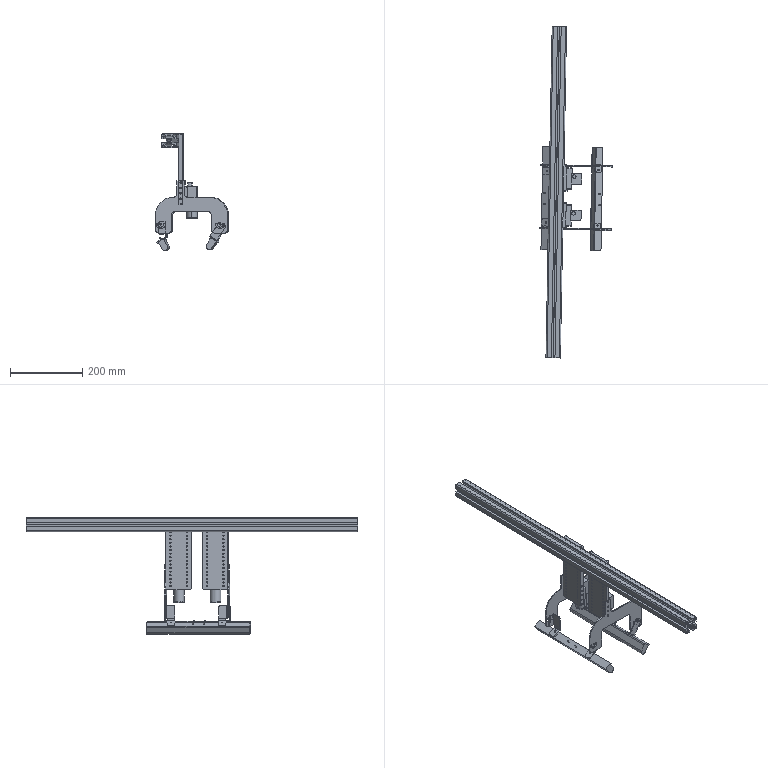Assembly | SolidWorks | mm | 17 component files | 19 solids | 825 faces | box 203.3 x 920.59 x 324.08 mm | volume 1362567 mm3 | cylinder 457 | plane 308 | cone 60 | commonest cylinder face diameters 3.3 x192 4.3 x48 2 x36 10 x22 6 x16 4.5 x16 1.6 x16 20 x16
Bill of materials:
A6061-4040-L920_AluminumExtrusion | 1 | 6061 Alloy | Long straight prismatic bar with a square cross-section. All four faces have a slot running the full length. The profile is hollow, with a central bore and cavities in the corners.
DM17A08-02-002 | 1 |  | Thin flat plate with an arch or inverted-U outline. A narrow tab with a single row of four small holes rises from the top. Each leg end has a small hole surrounded by a curved slot.
DM17A08-02-003 | 2 |  | Bent flat-strip bracket with two legs at roughly a right angle. The short leg has one round hole and the long leg has two round holes near its end. The corners are rounded.
DM17A08-02-004 | 1 |  | Bent strip bracket with a tall upright leg and a short foot bent at an obtuse angle. The upright has two holes near its top. The foot has one hole, and the upright edge has a stepped notch near the bend.
DM17A08-02-033 | 2 | 6061 Alloy | Elongated rectangular plate. Two long rows of small evenly spaced holes run along the face, with two larger holes near one end. A few small holes are on one long edge face, and the ends have raised lips.
DM17A08-04-008 | 2 | 6061 Alloy | Rectangular block. Two long slots run near opposite ends, and the central region has three round holes in a triangular pattern. The corners are chamfered and one face has a stepped rebate.
HikvisionCamera-MV-CA060-10GM | 2 | S45C | Square prism body with a small cylindrical boss on top and a larger cylindrical boss on the bottom. The bosses look coaxial or nearly so.
Lens | 2 | S45C | Solid stepped cylinder with three coaxial diameters. Going upward: a large main body, a slightly smaller short collar, then a small short boss.
LowerCameraLightSource | 2 | PP Copolymer | Long rectangular bar with two small cylindrical pins on one face near the middle. One end has a rounded or chamfered profile. A separate view shows a U-shaped section with a flange and a protruding pin.
Mirror_DM17A08-02-002 | 1 |  | Bent strip bracket with a tall upright leg and a short foot bent at an obtuse angle. The upright has two holes near its top. The foot has one hole, and the upright edge has a stepped notch near the bend.
Mirror_DM17A08-02-004 | 1 |  | Thin flat plate with an arch or inverted-U outline. A narrow tab with a single row of four small holes rises from the top. Each leg end has a small hole surrounded by a curved slot.
Mates:
1. concentric | HikvisionCamera-MV-CA060-10GM-1 face at (539.955, 339.268, 1015.886) dir (0, 0, 1) r 13 | Lens-1 face at (539.955, 339.268, 1020.386) dir (0, 0, -1) r 12.7
2. coincident | HikvisionCamera-MV-CA060-10GM-1 face at (539.955, 339.268, 1015.886) dir (0, 0, -1) | Lens-1 face at (539.955, 339.268, 1015.886) dir (0, 0, 1)
3. coincident | DM17A08-02-033-1 face at (512.46, 339.783, 1115.565) dir (0.9998, -0.01873, 0) | DM17A08-04-008-1 face at (512.46, 339.783, 1046.565) dir (-0.9998, 0.01873, 0)
4. coincident | DM17A08-02-033-1 face at (513.022, 369.778, 1215.565) dir (-0.01873, -0.9998, 0) | DM17A08-04-008-1 face at (528.019, 369.497, 1067.565) dir (0.01873, 0.9998, 0)
5. distance | DM17A08-04-008-1 face at (526.895, 309.507, 1025.565) dir (0, 0, -1) | DM17A08-02-033-1 face at (513.804, 304.752, 1015.565) dir (0, 0, -1)
6. coincident | DM17A08-02-033-1 face at (513.804, 304.752, 1215.565) dir (0, 0, 1) | A6061-4040-L920_AluminumExtrusion-1 face at (511.283, 864.223, 1215.565) dir (0, 0, 1)
7. coincident | DM17A08-02-033-1 face at (512.46, 339.783, 1115.565) dir (0.9998, -0.01873, 0) | DM17A08-02-033-2 face at (514.369, 441.679, 1115.565) dir (0.9998, -0.01873, 0)
8. coincident | DM17A08-04-008-1 face at (525.458, 339.539, 1046.565) dir (0.9998, -0.01873, 0) | HikvisionCamera-MV-CA060-10GM-1 face at (525.186, 325.042, 1069.565) dir (-0.9998, 0.01873, 0)
9. coincident | DM17A08-04-008-1 face at (525.186, 325.042, 1067.565) dir (0.01873, 0.9998, 0) | HikvisionCamera-MV-CA060-10GM-1 face at (554.181, 324.499, 1069.565) dir (-0.01873, -0.9998, 0)
10. distance | HikvisionCamera-MV-CA060-10GM-1 face at (539.955, 339.268, 1027.565) dir (0, 0, -1) | DM17A08-04-008-1 face at (526.895, 309.507, 1025.565) dir (0, 0, -1)
11. coincident | HikvisionCamera-MV-CA060-10GM-1 face at (539.955, 339.268, 1069.565) dir (0, 0, 1) | HikvisionCamera-MV-CA060-10GM-2 face at (541.864, 441.164, 1069.565) dir (0, 0, 1)
12. concentric | HikvisionCamera-MV-CA060-10GM-2 face at (541.864, 441.164, 1015.886) dir (0, 0, 1) r 13 | Lens-2 face at (541.864, 441.164, 1020.386) dir (0, 0, -1) r 12.7
13. coincident | HikvisionCamera-MV-CA060-10GM-2 face at (541.864, 441.164, 1015.886) dir (0, 0, -1) | Lens-2 face at (541.864, 441.164, 1015.886) dir (0, 0, 1)
14. coincident | DM17A08-02-033-2 face at (514.369, 441.679, 1115.565) dir (0.9998, -0.01873, 0) | DM17A08-04-008-2 face at (514.369, 441.679, 1046.565) dir (-0.9998, 0.01873, 0)
15. coincident | DM17A08-02-033-2 face at (514.931, 471.674, 1215.565) dir (-0.01873, -0.9998, 0) | DM17A08-04-008-2 face at (529.928, 471.393, 1067.565) dir (0.01873, 0.9998, 0)
16. distance | DM17A08-04-008-2 face at (528.804, 411.404, 1025.565) dir (0, 0, -1) | DM17A08-02-033-2 face at (515.713, 406.648, 1015.565) dir (0, 0, -1)
17. coincident | DM17A08-02-033-2 face at (517.024, 476.636, 1215.565) dir (0.01873, 0.9998, 0) | DM17A08-02-002-1 face at (522.023, 476.542, 1039.161) dir (-0.01873, -0.9998, 0)
18. width | DM17A08-02-033-2 face at (516.369, 441.642, 1115.565) dir (0.9998, -0.01873, 0) | DM17A08-02-033-2 face at (506.37, 441.829, 1115.565) dir (-0.9998, 0.01873, 0) | DM17A08-02-002-1 face at (502.083, 479.916, 1084.994) dir (-0.9998, 0.01873, 0) | DM17A08-02-002-1 face at (522.08, 479.541, 1039.161) dir (0.9998, -0.01873, 0)
19. coincident | DM17A08-04-008-2 face at (527.367, 441.436, 1046.565) dir (0.9998, -0.01873, 0) | HikvisionCamera-MV-CA060-10GM-2 face at (527.095, 426.938, 1069.565) dir (-0.9998, 0.01873, 0)
20. coincident | DM17A08-04-008-2 face at (527.095, 426.938, 1067.565) dir (0.01873, 0.9998, 0) | HikvisionCamera-MV-CA060-10GM-2 face at (556.09, 426.395, 1069.565) dir (-0.01873, -0.9998, 0)
21. distance | HikvisionCamera-MV-CA060-10GM-2 face at (541.864, 441.164, 1027.565) dir (0, 0, -1) | DM17A08-04-008-2 face at (528.804, 411.404, 1025.565) dir (0, 0, -1)
22. parallel | HikvisionCamera-MV-CA060-10GM-2 edge at (556.09, 426.395, 1069.565) dir (0.01873, 0.9998, 0) | LowerCameraLightSource-1 edge at (609.632, 242.152, 915.9) dir (0.01873, 0.9998, 0)
23. parallel | HikvisionCamera-MV-CA060-10GM-2 face at (556.09, 426.395, 1069.565) dir (0.9998, -0.01873, 0) | LowerCameraLightSource-2 edge at (462.203, 244.916, 924.969) dir (0.01873, 0.9998, 0)
24. coincident | DM17A08-02-002-1 face at (522.023, 476.542, 1039.161) dir (-0.01873, -0.9998, 0) | DM17A08-02-004-1 face at (451.607, 477.861, 971.563) dir (0.01873, 0.9998, 0)
25. concentric | DM17A08-02-002-1 face at (622.006, 474.669, 964.161) dir (-0.01873, -0.9998, 0) r 2.15 | DM17A08-02-003-1 face at (622.062, 477.668, 964.161) dir (-0.01873, -0.9998, 0) r 2.15